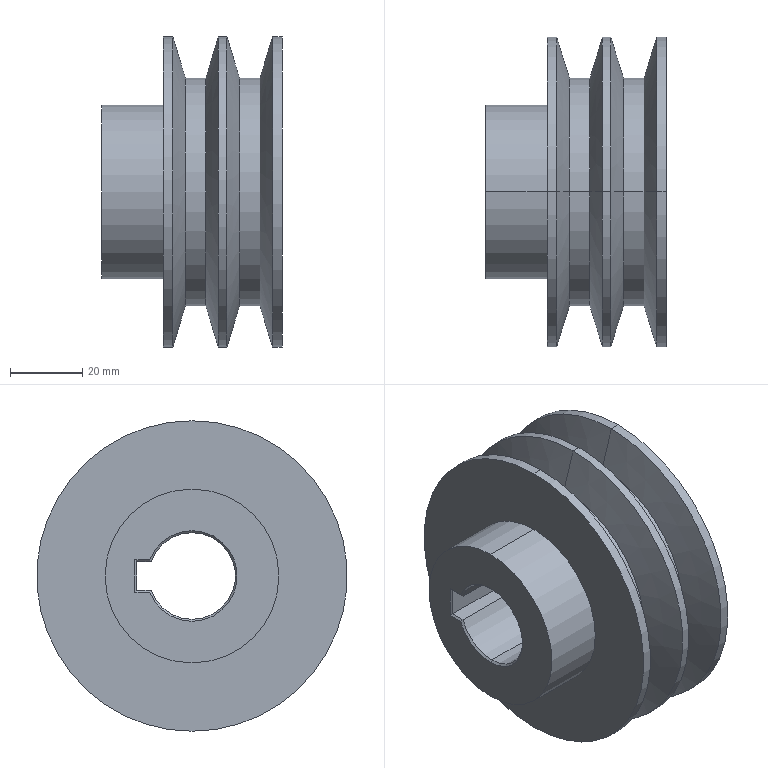Component | SolidWorks | V-beltSmallSolidWheel86x24.075x48-1 | 1 solid | 41 faces | box 50 x 86 x 86 mm | volume 148389 mm3 | cylinder 15 | cone 14 | plane 12 | commonest cylinder face diameters 86 x6 63.1 x4 24 x3 48.15 x2 | material Plain Carbon Steel
STEP:
#1=COLOUR_RGB('',0.7922,0.8196,0.9333);
#2=FILL_AREA_STYLE_COLOUR('',#1);
#3=FILL_AREA_STYLE('',(#2));
#4=SURFACE_STYLE_FILL_AREA(#3);
#5=SURFACE_SIDE_STYLE('',(#4));
#6=SURFACE_STYLE_USAGE(.BOTH.,#5);
#7=PRESENTATION_STYLE_ASSIGNMENT((#6));
#8=CARTESIAN_POINT('',(-20.311,-5.118,17.803));
#9=VERTEX_POINT('',#8);
#10=CARTESIAN_POINT('',(-20.311,-5.118,16.858));
#11=VERTEX_POINT('',#10);
#12=CARTESIAN_POINT('',(-20.311,-5.118,17.331));
#13=DIRECTION('',(1.,0.,-0.));
#14=DIRECTION('',(0.,0.,1.));
#15=AXIS2_PLACEMENT_3D('',#12,#13,#14);
#16=CIRCLE('',#15,0.4724);
#17=EDGE_CURVE('',#9,#11,#16,.T.);
#18=ORIENTED_EDGE('',*,*,#17,.F.);
#19=CARTESIAN_POINT('',(-20.29,-5.118,17.825));
#20=VERTEX_POINT('',#19);
#21=CARTESIAN_POINT('',(-20.311,-5.118,17.803));
#22=DIRECTION('',(0.7071,0.,0.7071));
#23=VECTOR('',#22,39.37);
#24=LINE('',#21,#23);
#25=EDGE_CURVE('',#9,#20,#24,.T.);
#26=ORIENTED_EDGE('',*,*,#25,.T.);
#27=CARTESIAN_POINT('',(-20.29,-5.118,16.837));
#28=VERTEX_POINT('',#27);
#29=CARTESIAN_POINT('',(-20.29,-5.118,17.331));
#30=DIRECTION('',(-1.,-0.,0.));
#31=DIRECTION('',(0.,0.,1.));
#32=AXIS2_PLACEMENT_3D('',#29,#30,#31);
#33=CIRCLE('',#32,0.4939);
#34=EDGE_CURVE('',#28,#20,#33,.T.);
#35=ORIENTED_EDGE('',*,*,#34,.F.);
#36=CARTESIAN_POINT('',(-20.311,-5.118,16.858));
#37=DIRECTION('',(0.7071,0.,-0.7071));
#38=VECTOR('',#37,39.37);
#39=LINE('',#36,#38);
#40=EDGE_CURVE('',#11,#28,#39,.T.);
#41=ORIENTED_EDGE('',*,*,#40,.F.);
#42=EDGE_LOOP('',(#18,#26,#35,#41));
#43=FACE_OUTER_BOUND('',#42,.T.);
#44=CARTESIAN_POINT('',(-20.311,-5.118,17.331));
#45=DIRECTION('',(1.,0.,-0.));
#46=DIRECTION('',(0.,0.,-1.));
#47=AXIS2_PLACEMENT_3D('',#44,#45,#46);
#48=CONICAL_SURFACE('',#47,0.4724,0.7854);
#49=ADVANCED_FACE('',(#43),#48,.F.);
#50=CARTESIAN_POINT('',(-20.311,-4.673,17.173));
#51=VERTEX_POINT('',#50);
#52=CARTESIAN_POINT('',(-20.311,-5.118,17.331));
#53=DIRECTION('',(1.,0.,-0.));
#54=DIRECTION('',(0.,0.,1.));
#55=AXIS2_PLACEMENT_3D('',#52,#53,#54);
#56=CIRCLE('',#55,0.4724);
#57=EDGE_CURVE('',#11,#51,#56,.T.);
#58=ORIENTED_EDGE('',*,*,#57,.F.);
#59=ORIENTED_EDGE('',*,*,#40,.T.);
#60=CARTESIAN_POINT('',(-20.29,-4.658,17.152));
#61=VERTEX_POINT('',#60);
#62=CARTESIAN_POINT('',(-20.29,-5.118,17.331));
#63=DIRECTION('',(-1.,-0.,0.));
#64=DIRECTION('',(0.,0.,1.));
#65=AXIS2_PLACEMENT_3D('',#62,#63,#64);
#66=CIRCLE('',#65,0.4939);
#67=EDGE_CURVE('',#61,#28,#66,.T.);
#68=ORIENTED_EDGE('',*,*,#67,.F.);
#69=CARTESIAN_POINT('',(-20.311,-4.673,17.173));
#70=CARTESIAN_POINT('',(-20.304,-4.668,17.166));
#71=CARTESIAN_POINT('',(-20.297,-4.663,17.159));
#72=CARTESIAN_POINT('',(-20.29,-4.658,17.152));
#73=B_SPLINE_CURVE_WITH_KNOTS('',3,(#69,#70,#71,#72),.UNSPECIFIED.,.F.,.F.,(4,4),(0.,0.0008589),.UNSPECIFIED.);
#74=EDGE_CURVE('',#51,#61,#73,.T.);
#75=ORIENTED_EDGE('',*,*,#74,.F.);
#76=EDGE_LOOP('',(#58,#59,#68,#75));
#77=FACE_OUTER_BOUND('',#76,.T.);
#78=CARTESIAN_POINT('',(-20.311,-5.118,17.331));
#79=DIRECTION('',(1.,0.,-0.));
#80=DIRECTION('',(0.,0.,-1.));
#81=AXIS2_PLACEMENT_3D('',#78,#79,#80);
#82=CONICAL_SURFACE('',#81,0.4724,0.7854);
#83=ADVANCED_FACE('',(#77),#82,.F.);
#84=CARTESIAN_POINT('',(-22.237,-5.118,16.858));
#85=VERTEX_POINT('',#84);
#86=CARTESIAN_POINT('',(-22.237,-5.118,17.803));
#87=VERTEX_POINT('',#86);
#88=CARTESIAN_POINT('',(-22.237,-5.118,17.331));
#89=DIRECTION('',(-1.,-0.,0.));
#90=DIRECTION('',(0.,0.,-1.));
#91=AXIS2_PLACEMENT_3D('',#88,#89,#90);
#92=CIRCLE('',#91,0.4724);
#93=EDGE_CURVE('',#85,#87,#92,.T.);
#94=ORIENTED_EDGE('',*,*,#93,.F.);
#95=CARTESIAN_POINT('',(-22.258,-5.118,16.837));
#96=VERTEX_POINT('',#95);
#97=CARTESIAN_POINT('',(-22.258,-5.118,16.837));
#98=DIRECTION('',(-0.7071,0.,-0.7071));
#99=VECTOR('',#98,39.37);
#100=LINE('',#97,#99);
#101=EDGE_CURVE('',#85,#96,#100,.T.);
#102=ORIENTED_EDGE('',*,*,#101,.T.);
#103=CARTESIAN_POINT('',(-22.258,-5.118,17.825));
#104=VERTEX_POINT('',#103);
#105=CARTESIAN_POINT('',(-22.258,-5.118,17.331));
#106=DIRECTION('',(1.,0.,-0.));
#107=DIRECTION('',(0.,0.,-1.));
#108=AXIS2_PLACEMENT_3D('',#105,#106,#107);
#109=CIRCLE('',#108,0.4939);
#110=EDGE_CURVE('',#104,#96,#109,.T.);
#111=ORIENTED_EDGE('',*,*,#110,.F.);
#112=CARTESIAN_POINT('',(-22.258,-5.118,17.825));
#113=DIRECTION('',(-0.7071,-0.,0.7071));
#114=VECTOR('',#113,39.37);
#115=LINE('',#112,#114);
#116=EDGE_CURVE('',#87,#104,#115,.T.);
#117=ORIENTED_EDGE('',*,*,#116,.F.);
#118=EDGE_LOOP('',(#94,#102,#111,#117));
#119=FACE_OUTER_BOUND('',#118,.T.);
#120=CARTESIAN_POINT('',(-22.258,-5.118,17.331));
#121=DIRECTION('',(-1.,-0.,0.));
#122=DIRECTION('',(0.,0.,1.));
#123=AXIS2_PLACEMENT_3D('',#120,#121,#122);
#124=CONICAL_SURFACE('',#123,0.4939,0.7854);
#125=ADVANCED_FACE('',(#119),#124,.F.);
#126=CARTESIAN_POINT('',(-22.237,-4.673,17.488));
#127=VERTEX_POINT('',#126);
#128=CARTESIAN_POINT('',(-22.237,-5.118,17.331));
#129=DIRECTION('',(-1.,-0.,0.));
#130=DIRECTION('',(0.,0.,-1.));
#131=AXIS2_PLACEMENT_3D('',#128,#129,#130);
#132=CIRCLE('',#131,0.4724);
#133=EDGE_CURVE('',#87,#127,#132,.T.);
#134=ORIENTED_EDGE('',*,*,#133,.F.);
#135=ORIENTED_EDGE('',*,*,#116,.T.);
#136=CARTESIAN_POINT('',(-22.258,-4.658,17.51));
#137=VERTEX_POINT('',#136);
#138=CARTESIAN_POINT('',(-22.258,-5.118,17.331));
#139=DIRECTION('',(1.,0.,-0.));
#140=DIRECTION('',(0.,0.,-1.));
#141=AXIS2_PLACEMENT_3D('',#138,#139,#140);
#142=CIRCLE('',#141,0.4939);
#143=EDGE_CURVE('',#137,#104,#142,.T.);
#144=ORIENTED_EDGE('',*,*,#143,.F.);
#145=CARTESIAN_POINT('',(-22.237,-4.673,17.488));
#146=CARTESIAN_POINT('',(-22.244,-4.668,17.496));
#147=CARTESIAN_POINT('',(-22.251,-4.663,17.503));
#148=CARTESIAN_POINT('',(-22.258,-4.658,17.51));
#149=B_SPLINE_CURVE_WITH_KNOTS('',3,(#145,#146,#147,#148),.UNSPECIFIED.,.F.,.F.,(4,4),(0.,0.0008589),.UNSPECIFIED.);
#150=EDGE_CURVE('',#127,#137,#149,.T.);
#151=ORIENTED_EDGE('',*,*,#150,.F.);
#152=EDGE_LOOP('',(#134,#135,#144,#151));
#153=FACE_OUTER_BOUND('',#152,.T.);
#154=CARTESIAN_POINT('',(-22.258,-5.118,17.331));
#155=DIRECTION('',(-1.,-0.,0.));
#156=DIRECTION('',(0.,0.,1.));
#157=AXIS2_PLACEMENT_3D('',#154,#155,#156);
#158=CONICAL_SURFACE('',#157,0.4939,0.7854);
#159=ADVANCED_FACE('',(#153),#158,.F.);
#160=CARTESIAN_POINT('',(-21.123,-5.118,16.089));
#161=VERTEX_POINT('',#160);
#162=CARTESIAN_POINT('',(-21.123,-5.118,18.573));
#163=VERTEX_POINT('',#162);
#164=CARTESIAN_POINT('',(-21.123,-5.118,17.331));
#165=DIRECTION('',(1.,0.,-0.));
#166=DIRECTION('',(0.,0.,-1.));
#167=AXIS2_PLACEMENT_3D('',#164,#165,#166);
#168=CIRCLE('',#167,1.242);
#169=EDGE_CURVE('',#161,#163,#168,.T.);
#170=ORIENTED_EDGE('',*,*,#169,.T.);
#171=CARTESIAN_POINT('',(-20.985,-5.118,19.024));
#172=VERTEX_POINT('',#171);
#173=CARTESIAN_POINT('',(-20.985,-5.118,19.024));
#174=DIRECTION('',(0.2924,0.,0.9563));
#175=VECTOR('',#174,39.37);
#176=LINE('',#173,#175);
#177=EDGE_CURVE('',#163,#172,#176,.T.);
#178=ORIENTED_EDGE('',*,*,#177,.T.);
#179=CARTESIAN_POINT('',(-20.985,-5.118,15.638));
#180=VERTEX_POINT('',#179);
#181=CARTESIAN_POINT('',(-20.985,-5.118,17.331));
#182=DIRECTION('',(1.,0.,-0.));
#183=DIRECTION('',(0.,0.,-1.));
#184=AXIS2_PLACEMENT_3D('',#181,#182,#183);
#185=CIRCLE('',#184,1.693);
#186=EDGE_CURVE('',#180,#172,#185,.T.);
#187=ORIENTED_EDGE('',*,*,#186,.F.);
#188=CARTESIAN_POINT('',(-20.985,-5.118,15.638));
#189=DIRECTION('',(0.2924,0.,-0.9563));
#190=VECTOR('',#189,39.37);
#191=LINE('',#188,#190);
#192=EDGE_CURVE('',#161,#180,#191,.T.);
#193=ORIENTED_EDGE('',*,*,#192,.F.);
#194=EDGE_LOOP('',(#170,#178,#187,#193));
#195=FACE_OUTER_BOUND('',#194,.T.);
#196=CARTESIAN_POINT('',(-20.985,-5.118,17.331));
#197=DIRECTION('',(1.,0.,-0.));
#198=DIRECTION('',(0.,0.,-1.));
#199=AXIS2_PLACEMENT_3D('',#196,#197,#198);
#200=CONICAL_SURFACE('',#199,1.693,1.274);
#201=ADVANCED_FACE('',(#195),#200,.T.);
#202=CARTESIAN_POINT('',(-21.347,-5.118,16.089));
#203=VERTEX_POINT('',#202);
#204=CARTESIAN_POINT('',(-21.347,-5.118,18.573));
#205=VERTEX_POINT('',#204);
#206=CARTESIAN_POINT('',(-21.347,-5.118,17.331));
#207=DIRECTION('',(1.,0.,-0.));
#208=DIRECTION('',(0.,0.,-1.));
#209=AXIS2_PLACEMENT_3D('',#206,#207,#208);
#210=CIRCLE('',#209,1.242);
#211=EDGE_CURVE('',#203,#205,#210,.T.);
#212=ORIENTED_EDGE('',*,*,#211,.F.);
#213=CARTESIAN_POINT('',(-21.484,-5.118,15.638));
#214=VERTEX_POINT('',#213);
#215=CARTESIAN_POINT('',(-21.347,-5.118,16.089));
#216=DIRECTION('',(-0.2924,0.,-0.9563));
#217=VECTOR('',#216,39.37);
#218=LINE('',#215,#217);
#219=EDGE_CURVE('',#203,#214,#218,.T.);
#220=ORIENTED_EDGE('',*,*,#219,.T.);
#221=CARTESIAN_POINT('',(-21.484,-5.118,19.024));
#222=VERTEX_POINT('',#221);
#223=CARTESIAN_POINT('',(-21.484,-5.118,17.331));
#224=DIRECTION('',(1.,0.,-0.));
#225=DIRECTION('',(0.,0.,-1.));
#226=AXIS2_PLACEMENT_3D('',#223,#224,#225);
#227=CIRCLE('',#226,1.693);
#228=EDGE_CURVE('',#214,#222,#227,.T.);
#229=ORIENTED_EDGE('',*,*,#228,.T.);
#230=CARTESIAN_POINT('',(-21.347,-5.118,18.573));
#231=DIRECTION('',(-0.2924,-0.,0.9563));
#232=VECTOR('',#231,39.37);
#233=LINE('',#230,#232);
#234=EDGE_CURVE('',#205,#222,#233,.T.);
#235=ORIENTED_EDGE('',*,*,#234,.F.);
#236=EDGE_LOOP('',(#212,#220,#229,#235));
#237=FACE_OUTER_BOUND('',#236,.T.);
#238=CARTESIAN_POINT('',(-21.347,-5.118,17.331));
#239=DIRECTION('',(-1.,-0.,0.));
#240=DIRECTION('',(0.,0.,1.));
#241=AXIS2_PLACEMENT_3D('',#238,#239,#240);
#242=CONICAL_SURFACE('',#241,1.242,1.274);
#243=ADVANCED_FACE('',(#237),#242,.T.);
#244=ORIENTED_EDGE('',*,*,#211,.T.);
#245=CARTESIAN_POINT('',(-21.235,-5.118,18.573));
#246=DIRECTION('',(1.,0.,-0.));
#247=VECTOR('',#246,39.37);
#248=LINE('',#245,#247);
#249=EDGE_CURVE('',#205,#163,#248,.T.);
#250=ORIENTED_EDGE('',*,*,#249,.T.);
#251=ORIENTED_EDGE('',*,*,#169,.F.);
#252=CARTESIAN_POINT('',(-21.235,-5.118,16.089));
#253=DIRECTION('',(1.,0.,-0.));
#254=VECTOR('',#253,39.37);
#255=LINE('',#252,#254);
#256=EDGE_CURVE('',#203,#161,#255,.T.);
#257=ORIENTED_EDGE('',*,*,#256,.F.);
#258=EDGE_LOOP('',(#244,#250,#251,#257));
#259=FACE_OUTER_BOUND('',#258,.T.);
#260=CARTESIAN_POINT('',(-21.235,-5.118,17.331));
#261=DIRECTION('',(1.,0.,-0.));
#262=DIRECTION('',(0.,0.,-1.));
#263=AXIS2_PLACEMENT_3D('',#260,#261,#262);
#264=CYLINDRICAL_SURFACE('',#263,1.242);
#265=ADVANCED_FACE('',(#259),#264,.T.);
#266=CARTESIAN_POINT('',(-20.532,-5.118,16.089));
#267=VERTEX_POINT('',#266);
#268=CARTESIAN_POINT('',(-20.532,-5.118,18.573));
#269=VERTEX_POINT('',#268);
#270=CARTESIAN_POINT('',(-20.532,-5.118,17.331));
#271=DIRECTION('',(1.,0.,-0.));
#272=DIRECTION('',(0.,0.,-1.));
#273=AXIS2_PLACEMENT_3D('',#270,#271,#272);
#274=CIRCLE('',#273,1.242);
#275=EDGE_CURVE('',#267,#269,#274,.T.);
#276=ORIENTED_EDGE('',*,*,#275,.T.);
#277=CARTESIAN_POINT('',(-20.395,-5.118,19.024));
#278=VERTEX_POINT('',#277);
#279=CARTESIAN_POINT('',(-20.395,-5.118,19.024));
#280=DIRECTION('',(0.2924,0.,0.9563));
#281=VECTOR('',#280,39.37);
#282=LINE('',#279,#281);
#283=EDGE_CURVE('',#269,#278,#282,.T.);
#284=ORIENTED_EDGE('',*,*,#283,.T.);
#285=CARTESIAN_POINT('',(-20.395,-5.118,15.638));
#286=VERTEX_POINT('',#285);
#287=CARTESIAN_POINT('',(-20.395,-5.118,17.331));
#288=DIRECTION('',(1.,0.,-0.));
#289=DIRECTION('',(0.,0.,-1.));
#290=AXIS2_PLACEMENT_3D('',#287,#288,#289);
#291=CIRCLE('',#290,1.693);
#292=EDGE_CURVE('',#286,#278,#291,.T.);
#293=ORIENTED_EDGE('',*,*,#292,.F.);
#294=CARTESIAN_POINT('',(-20.395,-5.118,15.638));
#295=DIRECTION('',(0.2924,0.,-0.9563));
#296=VECTOR('',#295,39.37);
#297=LINE('',#294,#296);
#298=EDGE_CURVE('',#267,#286,#297,.T.);
#299=ORIENTED_EDGE('',*,*,#298,.F.);
#300=EDGE_LOOP('',(#276,#284,#293,#299));
#301=FACE_OUTER_BOUND('',#300,.T.);
#302=CARTESIAN_POINT('',(-20.395,-5.118,17.331));
#303=DIRECTION('',(1.,0.,-0.));
#304=DIRECTION('',(0.,0.,-1.));
#305=AXIS2_PLACEMENT_3D('',#302,#303,#304);
#306=CONICAL_SURFACE('',#305,1.693,1.274);
#307=ADVANCED_FACE('',(#301),#306,.T.);
#308=CARTESIAN_POINT('',(-20.756,-5.118,16.089));
#309=VERTEX_POINT('',#308);
#310=CARTESIAN_POINT('',(-20.756,-5.118,18.573));
#311=VERTEX_POINT('',#310);
#312=CARTESIAN_POINT('',(-20.756,-5.118,17.331));
#313=DIRECTION('',(1.,0.,-0.));
#314=DIRECTION('',(0.,0.,-1.));
#315=AXIS2_PLACEMENT_3D('',#312,#313,#314);
#316=CIRCLE('',#315,1.242);
#317=EDGE_CURVE('',#309,#311,#316,.T.);
#318=ORIENTED_EDGE('',*,*,#317,.F.);
#319=CARTESIAN_POINT('',(-20.894,-5.118,15.638));
#320=VERTEX_POINT('',#319);
#321=CARTESIAN_POINT('',(-20.756,-5.118,16.089));
#322=DIRECTION('',(-0.2924,0.,-0.9563));
#323=VECTOR('',#322,39.37);
#324=LINE('',#321,#323);
#325=EDGE_CURVE('',#309,#320,#324,.T.);
#326=ORIENTED_EDGE('',*,*,#325,.T.);
#327=CARTESIAN_POINT('',(-20.894,-5.118,19.024));
#328=VERTEX_POINT('',#327);
#329=CARTESIAN_POINT('',(-20.894,-5.118,17.331));
#330=DIRECTION('',(1.,0.,-0.));
#331=DIRECTION('',(0.,0.,-1.));
#332=AXIS2_PLACEMENT_3D('',#329,#330,#331);
#333=CIRCLE('',#332,1.693);
#334=EDGE_CURVE('',#320,#328,#333,.T.);
#335=ORIENTED_EDGE('',*,*,#334,.T.);
#336=CARTESIAN_POINT('',(-20.756,-5.118,18.573));
#337=DIRECTION('',(-0.2924,-0.,0.9563));
#338=VECTOR('',#337,39.37);
#339=LINE('',#336,#338);
#340=EDGE_CURVE('',#311,#328,#339,.T.);
#341=ORIENTED_EDGE('',*,*,#340,.F.);
#342=EDGE_LOOP('',(#318,#326,#335,#341));
#343=FACE_OUTER_BOUND('',#342,.T.);
#344=CARTESIAN_POINT('',(-20.756,-5.118,17.331));
#345=DIRECTION('',(-1.,-0.,0.));
#346=DIRECTION('',(0.,0.,1.));
#347=AXIS2_PLACEMENT_3D('',#344,#345,#346);
#348=CONICAL_SURFACE('',#347,1.242,1.274);
#349=ADVANCED_FACE('',(#343),#348,.T.);
#350=ORIENTED_EDGE('',*,*,#317,.T.);
#351=CARTESIAN_POINT('',(-20.644,-5.118,18.573));
#352=DIRECTION('',(1.,0.,-0.));
#353=VECTOR('',#352,39.37);
#354=LINE('',#351,#353);
#355=EDGE_CURVE('',#311,#269,#354,.T.);
#356=ORIENTED_EDGE('',*,*,#355,.T.);
#357=ORIENTED_EDGE('',*,*,#275,.F.);
#358=CARTESIAN_POINT('',(-20.644,-5.118,16.089));
#359=DIRECTION('',(1.,0.,-0.));
#360=VECTOR('',#359,39.37);
#361=LINE('',#358,#360);
#362=EDGE_CURVE('',#309,#267,#361,.T.);
#363=ORIENTED_EDGE('',*,*,#362,.F.);
#364=EDGE_LOOP('',(#350,#356,#357,#363));
#365=FACE_OUTER_BOUND('',#364,.T.);
#366=CARTESIAN_POINT('',(-20.644,-5.118,17.331));
#367=DIRECTION('',(1.,0.,-0.));
#368=DIRECTION('',(0.,0.,-1.));
#369=AXIS2_PLACEMENT_3D('',#366,#367,#368);
#370=CYLINDRICAL_SURFACE('',#369,1.242);
#371=ADVANCED_FACE('',(#365),#370,.T.);
#372=CARTESIAN_POINT('',(-22.258,-5.118,16.383));
#373=VERTEX_POINT('',#372);
#374=CARTESIAN_POINT('',(-22.258,-5.118,18.279));
#375=VERTEX_POINT('',#374);
#376=CARTESIAN_POINT('',(-22.258,-5.118,17.331));
#377=DIRECTION('',(1.,0.,-0.));
#378=DIRECTION('',(0.,0.,-1.));
#379=AXIS2_PLACEMENT_3D('',#376,#377,#378);
#380=CIRCLE('',#379,0.9478);
#381=EDGE_CURVE('',#373,#375,#380,.T.);
#382=ORIENTED_EDGE('',*,*,#381,.T.);
#383=CARTESIAN_POINT('',(-21.589,-5.118,18.279));
#384=VERTEX_POINT('',#383);
#385=CARTESIAN_POINT('',(-20.644,-5.118,18.279));
#386=DIRECTION('',(1.,0.,-0.));
#387=VECTOR('',#386,39.37);
#388=LINE('',#385,#387);
#389=EDGE_CURVE('',#375,#384,#388,.T.);
#390=ORIENTED_EDGE('',*,*,#389,.T.);
#391=CARTESIAN_POINT('',(-21.589,-5.118,16.383));
#392=VERTEX_POINT('',#391);
#393=CARTESIAN_POINT('',(-21.589,-5.118,17.331));
#394=DIRECTION('',(1.,0.,-0.));
#395=DIRECTION('',(0.,0.,-1.));
#396=AXIS2_PLACEMENT_3D('',#393,#394,#395);
#397=CIRCLE('',#396,0.9478);
#398=EDGE_CURVE('',#392,#384,#397,.T.);
#399=ORIENTED_EDGE('',*,*,#398,.F.);
#400=CARTESIAN_POINT('',(-20.644,-5.118,16.383));
#401=DIRECTION('',(1.,0.,-0.));
#402=VECTOR('',#401,39.37);
#403=LINE('',#400,#402);
#404=EDGE_CURVE('',#373,#392,#403,.T.);
#405=ORIENTED_EDGE('',*,*,#404,.F.);
#406=EDGE_LOOP('',(#382,#390,#399,#405));
#407=FACE_OUTER_BOUND('',#406,.T.);
#408=CARTESIAN_POINT('',(-20.644,-5.118,17.331));
#409=DIRECTION('',(1.,0.,-0.));
#410=DIRECTION('',(0.,0.,-1.));
#411=AXIS2_PLACEMENT_3D('',#408,#409,#410);
#412=CYLINDRICAL_SURFACE('',#411,0.9478);
#413=ADVANCED_FACE('',(#407),#412,.T.);
#414=ORIENTED_EDGE('',*,*,#93,.T.);
#415=CARTESIAN_POINT('',(-20.644,-5.118,17.803));
#416=DIRECTION('',(1.,0.,-0.));
#417=VECTOR('',#416,39.37);
#418=LINE('',#415,#417);
#419=EDGE_CURVE('',#87,#9,#418,.T.);
#420=ORIENTED_EDGE('',*,*,#419,.T.);
#421=ORIENTED_EDGE('',*,*,#17,.T.);
#422=CARTESIAN_POINT('',(-20.644,-5.118,16.858));
#423=DIRECTION('',(1.,0.,-0.));
#424=VECTOR('',#423,39.37);
#425=LINE('',#422,#424);
#426=EDGE_CURVE('',#85,#11,#425,.T.);
#427=ORIENTED_EDGE('',*,*,#426,.F.);
#428=EDGE_LOOP('',(#414,#420,#421,#427));
#429=FACE_OUTER_BOUND('',#428,.T.);
#430=CARTESIAN_POINT('',(-20.644,-5.118,17.331));
#431=DIRECTION('',(1.,0.,-0.));
#432=DIRECTION('',(0.,0.,-1.));
#433=AXIS2_PLACEMENT_3D('',#430,#431,#432);
#434=CYLINDRICAL_SURFACE('',#433,0.4724);
#435=ADVANCED_FACE('',(#429),#434,.F.);
#436=CARTESIAN_POINT('',(-22.237,-4.673,17.173));
#437=VERTEX_POINT('',#436);
#438=CARTESIAN_POINT('',(-22.237,-5.118,17.331));
#439=DIRECTION('',(-1.,-0.,0.));
#440=DIRECTION('',(0.,0.,-1.));
#441=AXIS2_PLACEMENT_3D('',#438,#439,#440);
#442=CIRCLE('',#441,0.4724);
#443=EDGE_CURVE('',#437,#85,#442,.T.);
#444=ORIENTED_EDGE('',*,*,#443,.T.);
#445=ORIENTED_EDGE('',*,*,#426,.T.);
#446=ORIENTED_EDGE('',*,*,#57,.T.);
#447=CARTESIAN_POINT('',(-22.258,-4.673,17.173));
#448=DIRECTION('',(1.,0.,-0.));
#449=VECTOR('',#448,39.37);
#450=LINE('',#447,#449);
#451=EDGE_CURVE('',#437,#51,#450,.T.);
#452=ORIENTED_EDGE('',*,*,#451,.F.);
#453=EDGE_LOOP('',(#444,#445,#446,#452));
#454=FACE_OUTER_BOUND('',#453,.T.);
#455=CARTESIAN_POINT('',(-20.644,-5.118,17.331));
#456=DIRECTION('',(1.,0.,-0.));
#457=DIRECTION('',(0.,0.,-1.));
#458=AXIS2_PLACEMENT_3D('',#455,#456,#457);
#459=CYLINDRICAL_SURFACE('',#458,0.4724);
#460=ADVANCED_FACE('',(#454),#459,.F.);
#461=ORIENTED_EDGE('',*,*,#292,.T.);
#462=CARTESIAN_POINT('',(-20.29,-5.118,19.024));
#463=VERTEX_POINT('',#462);
#464=CARTESIAN_POINT('',(-20.644,-5.118,19.024));
#465=DIRECTION('',(1.,0.,-0.));
#466=VECTOR('',#465,39.37);
#467=LINE('',#464,#466);
#468=EDGE_CURVE('',#278,#463,#467,.T.);
#469=ORIENTED_EDGE('',*,*,#468,.T.);
#470=CARTESIAN_POINT('',(-20.29,-5.118,15.638));
#471=VERTEX_POINT('',#470);
#472=CARTESIAN_POINT('',(-20.29,-5.118,17.331));
#473=DIRECTION('',(1.,0.,-0.));
#474=DIRECTION('',(0.,0.,-1.));
#475=AXIS2_PLACEMENT_3D('',#472,#473,#474);
#476=CIRCLE('',#475,1.693);
#477=EDGE_CURVE('',#471,#463,#476,.T.);
#478=ORIENTED_EDGE('',*,*,#477,.F.);
#479=CARTESIAN_POINT('',(-20.644,-5.118,15.638));
#480=DIRECTION('',(1.,0.,-0.));
#481=VECTOR('',#480,39.37);
#482=LINE('',#479,#481);
#483=EDGE_CURVE('',#286,#471,#482,.T.);
#484=ORIENTED_EDGE('',*,*,#483,.F.);
#485=EDGE_LOOP('',(#461,#469,#478,#484));
#486=FACE_OUTER_BOUND('',#485,.T.);
#487=CARTESIAN_POINT('',(-20.644,-5.118,17.331));
#488=DIRECTION('',(1.,0.,-0.));
#489=DIRECTION('',(0.,0.,-1.));
#490=AXIS2_PLACEMENT_3D('',#487,#488,#489);
#491=CYLINDRICAL_SURFACE('',#490,1.693);
#492=ADVANCED_FACE('',(#486),#491,.T.);
#493=ORIENTED_EDGE('',*,*,#186,.T.);
#494=CARTESIAN_POINT('',(-20.644,-5.118,19.024));
#495=DIRECTION('',(1.,0.,-0.));
#496=VECTOR('',#495,39.37);
#497=LINE('',#494,#496);
#498=EDGE_CURVE('',#172,#328,#497,.T.);
#499=ORIENTED_EDGE('',*,*,#498,.T.);
#500=ORIENTED_EDGE('',*,*,#334,.F.);
#501=CARTESIAN_POINT('',(-20.644,-5.118,15.638));
#502=DIRECTION('',(1.,0.,-0.));
#503=VECTOR('',#502,39.37);
#504=LINE('',#501,#503);
#505=EDGE_CURVE('',#180,#320,#504,.T.);
#506=ORIENTED_EDGE('',*,*,#505,.F.);
#507=EDGE_LOOP('',(#493,#499,#500,#506));
#508=FACE_OUTER_BOUND('',#507,.T.);
#509=CARTESIAN_POINT('',(-20.644,-5.118,17.331));
#510=DIRECTION('',(1.,0.,-0.));
#511=DIRECTION('',(0.,0.,-1.));
#512=AXIS2_PLACEMENT_3D('',#509,#510,#511);
#513=CYLINDRICAL_SURFACE('',#512,1.693);
#514=ADVANCED_FACE('',(#508),#513,.T.);
#515=CARTESIAN_POINT('',(-21.589,-5.118,15.638));
#516=VERTEX_POINT('',#515);
#517=CARTESIAN_POINT('',(-21.589,-5.118,19.024));
#518=VERTEX_POINT('',#517);
#519=CARTESIAN_POINT('',(-21.589,-5.118,17.331));
#520=DIRECTION('',(1.,0.,-0.));
#521=DIRECTION('',(0.,0.,-1.));
#522=AXIS2_PLACEMENT_3D('',#519,#520,#521);
#523=CIRCLE('',#522,1.693);
#524=EDGE_CURVE('',#516,#518,#523,.T.);
#525=ORIENTED_EDGE('',*,*,#524,.T.);
#526=CARTESIAN_POINT('',(-20.644,-5.118,19.024));
#527=DIRECTION('',(1.,0.,-0.));
#528=VECTOR('',#527,39.37);
#529=LINE('',#526,#528);
#530=EDGE_CURVE('',#518,#222,#529,.T.);
#531=ORIENTED_EDGE('',*,*,#530,.T.);
#532=ORIENTED_EDGE('',*,*,#228,.F.);
#533=CARTESIAN_POINT('',(-20.644,-5.118,15.638));
#534=DIRECTION('',(1.,0.,-0.));
#535=VECTOR('',#534,39.37);
#536=LINE('',#533,#535);
#537=EDGE_CURVE('',#516,#214,#536,.T.);
#538=ORIENTED_EDGE('',*,*,#537,.F.);
#539=EDGE_LOOP('',(#525,#531,#532,#538));
#540=FACE_OUTER_BOUND('',#539,.T.);
#541=CARTESIAN_POINT('',(-20.644,-5.118,17.331));
#542=DIRECTION('',(1.,0.,-0.));
#543=DIRECTION('',(0.,0.,-1.));
#544=AXIS2_PLACEMENT_3D('',#541,#542,#543);
#545=CYLINDRICAL_SURFACE('',#544,1.693);
#546=ADVANCED_FACE('',(#540),#545,.T.);
#547=ORIENTED_EDGE('',*,*,#530,.F.);
#548=CARTESIAN_POINT('',(-21.589,-5.118,17.331));
#549=DIRECTION('',(1.,0.,-0.));
#550=DIRECTION('',(0.,0.,-1.));
#551=AXIS2_PLACEMENT_3D('',#548,#549,#550);
#552=CIRCLE('',#551,1.693);
#553=EDGE_CURVE('',#518,#516,#552,.T.);
#554=ORIENTED_EDGE('',*,*,#553,.T.);
#555=ORIENTED_EDGE('',*,*,#537,.T.);
#556=CARTESIAN_POINT('',(-21.484,-5.118,17.331));
#557=DIRECTION('',(1.,0.,-0.));
#558=DIRECTION('',(0.,0.,-1.));
#559=AXIS2_PLACEMENT_3D('',#556,#557,#558);
#560=CIRCLE('',#559,1.693);
#561=EDGE_CURVE('',#222,#214,#560,.T.);
#562=ORIENTED_EDGE('',*,*,#561,.F.);
#563=EDGE_LOOP('',(#547,#554,#555,#562));
#564=FACE_OUTER_BOUND('',#563,.T.);
#565=CARTESIAN_POINT('',(-20.644,-5.118,17.331));
#566=DIRECTION('',(1.,0.,-0.));
#567=DIRECTION('',(0.,0.,-1.));
#568=AXIS2_PLACEMENT_3D('',#565,#566,#567);
#569=CYLINDRICAL_SURFACE('',#568,1.693);
#570=ADVANCED_FACE('',(#564),#569,.T.);
#571=ORIENTED_EDGE('',*,*,#498,.F.);
#572=CARTESIAN_POINT('',(-20.985,-5.118,17.331));
#573=DIRECTION('',(1.,0.,-0.));
#574=DIRECTION('',(0.,0.,-1.));
#575=AXIS2_PLACEMENT_3D('',#572,#573,#574);
#576=CIRCLE('',#575,1.693);
#577=EDGE_CURVE('',#172,#180,#576,.T.);
#578=ORIENTED_EDGE('',*,*,#577,.T.);
#579=ORIENTED_EDGE('',*,*,#505,.T.);
#580=CARTESIAN_POINT('',(-20.894,-5.118,17.331));
#581=DIRECTION('',(1.,0.,-0.));
#582=DIRECTION('',(0.,0.,-1.));
#583=AXIS2_PLACEMENT_3D('',#580,#581,#582);
#584=CIRCLE('',#583,1.693);
#585=EDGE_CURVE('',#328,#320,#584,.T.);
#586=ORIENTED_EDGE('',*,*,#585,.F.);
#587=EDGE_LOOP('',(#571,#578,#579,#586));
#588=FACE_OUTER_BOUND('',#587,.T.);
#589=CARTESIAN_POINT('',(-20.644,-5.118,17.331));
#590=DIRECTION('',(1.,0.,-0.));
#591=DIRECTION('',(0.,0.,-1.));
#592=AXIS2_PLACEMENT_3D('',#589,#590,#591);
#593=CYLINDRICAL_SURFACE('',#592,1.693);
#594=ADVANCED_FACE('',(#588),#593,.T.);
#595=ORIENTED_EDGE('',*,*,#468,.F.);
#596=CARTESIAN_POINT('',(-20.395,-5.118,17.331));
#597=DIRECTION('',(1.,0.,-0.));
#598=DIRECTION('',(0.,0.,-1.));
#599=AXIS2_PLACEMENT_3D('',#596,#597,#598);
#600=CIRCLE('',#599,1.693);
#601=EDGE_CURVE('',#278,#286,#600,.T.);
#602=ORIENTED_EDGE('',*,*,#601,.T.);
#603=ORIENTED_EDGE('',*,*,#483,.T.);
#604=CARTESIAN_POINT('',(-20.29,-5.118,17.331));
#605=DIRECTION('',(1.,0.,-0.));
#606=DIRECTION('',(0.,0.,-1.));
#607=AXIS2_PLACEMENT_3D('',#604,#605,#606);
#608=CIRCLE('',#607,1.693);
#609=EDGE_CURVE('',#463,#471,#608,.T.);
#610=ORIENTED_EDGE('',*,*,#609,.F.);
#611=EDGE_LOOP('',(#595,#602,#603,#610));
#612=FACE_OUTER_BOUND('',#611,.T.);
#613=CARTESIAN_POINT('',(-20.644,-5.118,17.331));
#614=DIRECTION('',(1.,0.,-0.));
#615=DIRECTION('',(0.,0.,-1.));
#616=AXIS2_PLACEMENT_3D('',#613,#614,#615);
#617=CYLINDRICAL_SURFACE('',#616,1.693);
#618=ADVANCED_FACE('',(#612),#617,.T.);
#619=ORIENTED_EDGE('',*,*,#419,.F.);
#620=ORIENTED_EDGE('',*,*,#133,.T.);
#621=CARTESIAN_POINT('',(-20.311,-4.673,17.488));
#622=VERTEX_POINT('',#621);
#623=CARTESIAN_POINT('',(-22.258,-4.673,17.488));
#624=DIRECTION('',(1.,0.,-0.));
#625=VECTOR('',#624,39.37);
#626=LINE('',#623,#625);
#627=EDGE_CURVE('',#127,#622,#626,.T.);
#628=ORIENTED_EDGE('',*,*,#627,.T.);
#629=CARTESIAN_POINT('',(-20.311,-5.118,17.331));
#630=DIRECTION('',(1.,0.,-0.));
#631=DIRECTION('',(0.,0.,1.));
#632=AXIS2_PLACEMENT_3D('',#629,#630,#631);
#633=CIRCLE('',#632,0.4724);
#634=EDGE_CURVE('',#622,#9,#633,.T.);
#635=ORIENTED_EDGE('',*,*,#634,.T.);
#636=EDGE_LOOP('',(#619,#620,#628,#635));
#637=FACE_OUTER_BOUND('',#636,.T.);
#638=CARTESIAN_POINT('',(-20.644,-5.118,17.331));
#639=DIRECTION('',(1.,0.,-0.));
#640=DIRECTION('',(0.,0.,-1.));
#641=AXIS2_PLACEMENT_3D('',#638,#639,#640);
#642=CYLINDRICAL_SURFACE('',#641,0.4724);
#643=ADVANCED_FACE('',(#637),#642,.F.);
#644=CARTESIAN_POINT('',(-22.258,-4.494,17.152));
#645=VERTEX_POINT('',#644);
#646=CARTESIAN_POINT('',(-22.258,-4.494,17.51));
#647=VERTEX_POINT('',#646);
#648=CARTESIAN_POINT('',(-22.258,-4.494,17.331));
#649=DIRECTION('',(0.,0.,1.));
#650=VECTOR('',#649,39.37);
#651=LINE('',#648,#650);
#652=EDGE_CURVE('',#645,#647,#651,.T.);
#653=ORIENTED_EDGE('',*,*,#652,.T.);
#654=CARTESIAN_POINT('',(-22.258,-4.17,17.51));
#655=DIRECTION('',(0.,-1.,0.));
#656=VECTOR('',#655,39.37);
#657=LINE('',#654,#656);
#658=EDGE_CURVE('',#647,#137,#657,.T.);
#659=ORIENTED_EDGE('',*,*,#658,.T.);
#660=ORIENTED_EDGE('',*,*,#143,.T.);
#661=ORIENTED_EDGE('',*,*,#110,.T.);
#662=CARTESIAN_POINT('',(-22.258,-4.658,17.152));
#663=VERTEX_POINT('',#662);
#664=CARTESIAN_POINT('',(-22.258,-5.118,17.331));
#665=DIRECTION('',(1.,0.,-0.));
#666=DIRECTION('',(0.,0.,-1.));
#667=AXIS2_PLACEMENT_3D('',#664,#665,#666);
#668=CIRCLE('',#667,0.4939);
#669=EDGE_CURVE('',#96,#663,#668,.T.);
#670=ORIENTED_EDGE('',*,*,#669,.T.);
#671=CARTESIAN_POINT('',(-22.258,-4.17,17.152));
#672=DIRECTION('',(-0.,1.,0.));
#673=VECTOR('',#672,39.37);
#674=LINE('',#671,#673);
#675=EDGE_CURVE('',#663,#645,#674,.T.);
#676=ORIENTED_EDGE('',*,*,#675,.T.);
#677=EDGE_LOOP('',(#653,#659,#660,#661,#670,#676));
#678=FACE_BOUND('',#677,.T.);
#679=ORIENTED_EDGE('',*,*,#381,.F.);
#680=CARTESIAN_POINT('',(-22.258,-5.118,17.331));
#681=DIRECTION('',(1.,0.,-0.));
#682=DIRECTION('',(0.,0.,-1.));
#683=AXIS2_PLACEMENT_3D('',#680,#681,#682);
#684=CIRCLE('',#683,0.9478);
#685=EDGE_CURVE('',#375,#373,#684,.T.);
#686=ORIENTED_EDGE('',*,*,#685,.F.);
#687=EDGE_LOOP('',(#679,#686));
#688=FACE_OUTER_BOUND('',#687,.T.);
#689=CARTESIAN_POINT('',(-22.258,-4.17,17.331));
#690=DIRECTION('',(1.,0.,-0.));
#691=DIRECTION('',(-0.,0.,-1.));
#692=AXIS2_PLACEMENT_3D('',#689,#690,#691);
#693=PLANE('',#692);
#694=ADVANCED_FACE('',(#678,#688),#693,.F.);
#695=ORIENTED_EDGE('',*,*,#389,.F.);
#696=ORIENTED_EDGE('',*,*,#685,.T.);
#697=ORIENTED_EDGE('',*,*,#404,.T.);
#698=CARTESIAN_POINT('',(-21.589,-5.118,17.331));
#699=DIRECTION('',(1.,0.,-0.));
#700=DIRECTION('',(0.,0.,-1.));
#701=AXIS2_PLACEMENT_3D('',#698,#699,#700);
#702=CIRCLE('',#701,0.9478);
#703=EDGE_CURVE('',#384,#392,#702,.T.);
#704=ORIENTED_EDGE('',*,*,#703,.F.);
#705=EDGE_LOOP('',(#695,#696,#697,#704));
#706=FACE_OUTER_BOUND('',#705,.T.);
#707=CARTESIAN_POINT('',(-20.644,-5.118,17.331));
#708=DIRECTION('',(1.,0.,-0.));
#709=DIRECTION('',(0.,0.,-1.));
#710=AXIS2_PLACEMENT_3D('',#707,#708,#709);
#711=CYLINDRICAL_SURFACE('',#710,0.9478);
#712=ADVANCED_FACE('',(#706),#711,.T.);
#713=ORIENTED_EDGE('',*,*,#524,.F.);
#714=ORIENTED_EDGE('',*,*,#553,.F.);
#715=EDGE_LOOP('',(#713,#714));
#716=FACE_OUTER_BOUND('',#715,.T.);
#717=ORIENTED_EDGE('',*,*,#398,.T.);
#718=ORIENTED_EDGE('',*,*,#703,.T.);
#719=EDGE_LOOP('',(#717,#718));
#720=FACE_BOUND('',#719,.T.);
#721=CARTESIAN_POINT('',(-21.589,-3.425,17.331));
#722=DIRECTION('',(1.,0.,-0.));
#723=DIRECTION('',(-0.,0.,-1.));
#724=AXIS2_PLACEMENT_3D('',#721,#722,#723);
#725=PLANE('',#724);
#726=ADVANCED_FACE('',(#716,#720),#725,.F.);
#727=CARTESIAN_POINT('',(-20.29,-4.494,17.51));
#728=VERTEX_POINT('',#727);
#729=CARTESIAN_POINT('',(-20.29,-4.494,17.152));
#730=VERTEX_POINT('',#729);
#731=CARTESIAN_POINT('',(-20.29,-4.494,17.331));
#732=DIRECTION('',(-0.,0.,-1.));
#733=VECTOR('',#732,39.37);
#734=LINE('',#731,#733);
#735=EDGE_CURVE('',#728,#730,#734,.T.);
#736=ORIENTED_EDGE('',*,*,#735,.T.);
#737=CARTESIAN_POINT('',(-20.29,-4.646,17.152));
#738=DIRECTION('',(0.,-1.,0.));
#739=VECTOR('',#738,39.37);
#740=LINE('',#737,#739);
#741=EDGE_CURVE('',#730,#61,#740,.T.);
#742=ORIENTED_EDGE('',*,*,#741,.T.);
#743=ORIENTED_EDGE('',*,*,#67,.T.);
#744=ORIENTED_EDGE('',*,*,#34,.T.);
#745=CARTESIAN_POINT('',(-20.29,-4.658,17.51));
#746=VERTEX_POINT('',#745);
#747=CARTESIAN_POINT('',(-20.29,-5.118,17.331));
#748=DIRECTION('',(-1.,-0.,0.));
#749=DIRECTION('',(0.,0.,1.));
#750=AXIS2_PLACEMENT_3D('',#747,#748,#749);
#751=CIRCLE('',#750,0.4939);
#752=EDGE_CURVE('',#20,#746,#751,.T.);
#753=ORIENTED_EDGE('',*,*,#752,.T.);
#754=CARTESIAN_POINT('',(-20.29,-4.646,17.51));
#755=DIRECTION('',(-0.,1.,0.));
#756=VECTOR('',#755,39.37);
#757=LINE('',#754,#756);
#758=EDGE_CURVE('',#746,#728,#757,.T.);
#759=ORIENTED_EDGE('',*,*,#758,.T.);
#760=EDGE_LOOP('',(#736,#742,#743,#744,#753,#759));
#761=FACE_BOUND('',#760,.T.);
#762=ORIENTED_EDGE('',*,*,#477,.T.);
#763=ORIENTED_EDGE('',*,*,#609,.T.);
#764=EDGE_LOOP('',(#762,#763));
#765=FACE_OUTER_BOUND('',#764,.T.);
#766=CARTESIAN_POINT('',(-20.29,-4.646,17.331));
#767=DIRECTION('',(-1.,-0.,0.));
#768=DIRECTION('',(0.,0.,1.));
#769=AXIS2_PLACEMENT_3D('',#766,#767,#768);
#770=PLANE('',#769);
#771=ADVANCED_FACE('',(#761,#765),#770,.F.);
#772=ORIENTED_EDGE('',*,*,#355,.F.);
#773=CARTESIAN_POINT('',(-20.756,-5.118,17.331));
#774=DIRECTION('',(1.,0.,-0.));
#775=DIRECTION('',(0.,0.,-1.));
#776=AXIS2_PLACEMENT_3D('',#773,#774,#775);
#777=CIRCLE('',#776,1.242);
#778=EDGE_CURVE('',#311,#309,#777,.T.);
#779=ORIENTED_EDGE('',*,*,#778,.T.);
#780=ORIENTED_EDGE('',*,*,#362,.T.);
#781=CARTESIAN_POINT('',(-20.532,-5.118,17.331));
#782=DIRECTION('',(1.,0.,-0.));
#783=DIRECTION('',(0.,0.,-1.));
#784=AXIS2_PLACEMENT_3D('',#781,#782,#783);
#785=CIRCLE('',#784,1.242);
#786=EDGE_CURVE('',#269,#267,#785,.T.);
#787=ORIENTED_EDGE('',*,*,#786,.F.);
#788=EDGE_LOOP('',(#772,#779,#780,#787));
#789=FACE_OUTER_BOUND('',#788,.T.);
#790=CARTESIAN_POINT('',(-20.644,-5.118,17.331));
#791=DIRECTION('',(1.,0.,-0.));
#792=DIRECTION('',(0.,0.,-1.));
#793=AXIS2_PLACEMENT_3D('',#790,#791,#792);
#794=CYLINDRICAL_SURFACE('',#793,1.242);
#795=ADVANCED_FACE('',(#789),#794,.T.);
#796=ORIENTED_EDGE('',*,*,#325,.F.);
#797=ORIENTED_EDGE('',*,*,#778,.F.);
#798=ORIENTED_EDGE('',*,*,#340,.T.);
#799=ORIENTED_EDGE('',*,*,#585,.T.);
#800=EDGE_LOOP('',(#796,#797,#798,#799));
#801=FACE_OUTER_BOUND('',#800,.T.);
#802=CARTESIAN_POINT('',(-20.756,-5.118,17.331));
#803=DIRECTION('',(-1.,-0.,0.));
#804=DIRECTION('',(0.,0.,1.));
#805=AXIS2_PLACEMENT_3D('',#802,#803,#804);
#806=CONICAL_SURFACE('',#805,1.242,1.274);
#807=ADVANCED_FACE('',(#801),#806,.T.);
#808=ORIENTED_EDGE('',*,*,#283,.F.);
#809=ORIENTED_EDGE('',*,*,#786,.T.);
#810=ORIENTED_EDGE('',*,*,#298,.T.);
#811=ORIENTED_EDGE('',*,*,#601,.F.);
#812=EDGE_LOOP('',(#808,#809,#810,#811));
#813=FACE_OUTER_BOUND('',#812,.T.);
#814=CARTESIAN_POINT('',(-20.395,-5.118,17.331));
#815=DIRECTION('',(1.,0.,-0.));
#816=DIRECTION('',(0.,0.,-1.));
#817=AXIS2_PLACEMENT_3D('',#814,#815,#816);
#818=CONICAL_SURFACE('',#817,1.693,1.274);
#819=ADVANCED_FACE('',(#813),#818,.T.);
#820=ORIENTED_EDGE('',*,*,#249,.F.);
#821=CARTESIAN_POINT('',(-21.347,-5.118,17.331));
#822=DIRECTION('',(1.,0.,-0.));
#823=DIRECTION('',(0.,0.,-1.));
#824=AXIS2_PLACEMENT_3D('',#821,#822,#823);
#825=CIRCLE('',#824,1.242);
#826=EDGE_CURVE('',#205,#203,#825,.T.);
#827=ORIENTED_EDGE('',*,*,#826,.T.);
#828=ORIENTED_EDGE('',*,*,#256,.T.);
#829=CARTESIAN_POINT('',(-21.123,-5.118,17.331));
#830=DIRECTION('',(1.,0.,-0.));
#831=DIRECTION('',(0.,0.,-1.));
#832=AXIS2_PLACEMENT_3D('',#829,#830,#831);
#833=CIRCLE('',#832,1.242);
#834=EDGE_CURVE('',#163,#161,#833,.T.);
#835=ORIENTED_EDGE('',*,*,#834,.F.);
#836=EDGE_LOOP('',(#820,#827,#828,#835));
#837=FACE_OUTER_BOUND('',#836,.T.);
#838=CARTESIAN_POINT('',(-21.235,-5.118,17.331));
#839=DIRECTION('',(1.,0.,-0.));
#840=DIRECTION('',(0.,0.,-1.));
#841=AXIS2_PLACEMENT_3D('',#838,#839,#840);
#842=CYLINDRICAL_SURFACE('',#841,1.242);
#843=ADVANCED_FACE('',(#837),#842,.T.);
#844=ORIENTED_EDGE('',*,*,#219,.F.);
#845=ORIENTED_EDGE('',*,*,#826,.F.);
#846=ORIENTED_EDGE('',*,*,#234,.T.);
#847=ORIENTED_EDGE('',*,*,#561,.T.);
#848=EDGE_LOOP('',(#844,#845,#846,#847));
#849=FACE_OUTER_BOUND('',#848,.T.);
#850=CARTESIAN_POINT('',(-21.347,-5.118,17.331));
#851=DIRECTION('',(-1.,-0.,0.));
#852=DIRECTION('',(0.,0.,1.));
#853=AXIS2_PLACEMENT_3D('',#850,#851,#852);
#854=CONICAL_SURFACE('',#853,1.242,1.274);
#855=ADVANCED_FACE('',(#849),#854,.T.);
#856=ORIENTED_EDGE('',*,*,#177,.F.);
#857=ORIENTED_EDGE('',*,*,#834,.T.);
#858=ORIENTED_EDGE('',*,*,#192,.T.);
#859=ORIENTED_EDGE('',*,*,#577,.F.);
#860=EDGE_LOOP('',(#856,#857,#858,#859));
#861=FACE_OUTER_BOUND('',#860,.T.);
#862=CARTESIAN_POINT('',(-20.985,-5.118,17.331));
#863=DIRECTION('',(1.,0.,-0.));
#864=DIRECTION('',(0.,0.,-1.));
#865=AXIS2_PLACEMENT_3D('',#862,#863,#864);
#866=CONICAL_SURFACE('',#865,1.693,1.274);
#867=ADVANCED_FACE('',(#861),#866,.T.);
#868=ORIENTED_EDGE('',*,*,#627,.F.);
#869=CARTESIAN_POINT('',(-22.237,-4.516,17.488));
#870=VERTEX_POINT('',#869);
#871=CARTESIAN_POINT('',(-22.237,-4.673,17.488));
#872=DIRECTION('',(-0.,1.,0.));
#873=VECTOR('',#872,39.37);
#874=LINE('',#871,#873);
#875=EDGE_CURVE('',#127,#870,#874,.T.);
#876=ORIENTED_EDGE('',*,*,#875,.T.);
#877=CARTESIAN_POINT('',(-20.311,-4.516,17.488));
#878=VERTEX_POINT('',#877);
#879=CARTESIAN_POINT('',(-22.258,-4.516,17.488));
#880=DIRECTION('',(1.,0.,-0.));
#881=VECTOR('',#880,39.37);
#882=LINE('',#879,#881);
#883=EDGE_CURVE('',#870,#878,#882,.T.);
#884=ORIENTED_EDGE('',*,*,#883,.T.);
#885=CARTESIAN_POINT('',(-20.311,-4.673,17.488));
#886=DIRECTION('',(0.,-1.,0.));
#887=VECTOR('',#886,39.37);
#888=LINE('',#885,#887);
#889=EDGE_CURVE('',#878,#622,#888,.T.);
#890=ORIENTED_EDGE('',*,*,#889,.T.);
#891=EDGE_LOOP('',(#868,#876,#884,#890));
#892=FACE_OUTER_BOUND('',#891,.T.);
#893=CARTESIAN_POINT('',(-22.258,-4.673,17.488));
#894=DIRECTION('',(0.,-0.,1.));
#895=DIRECTION('',(1.,0.,-0.));
#896=AXIS2_PLACEMENT_3D('',#893,#894,#895);
#897=PLANE('',#896);
#898=ADVANCED_FACE('',(#892),#897,.F.);
#899=ORIENTED_EDGE('',*,*,#883,.F.);
#900=CARTESIAN_POINT('',(-22.237,-4.516,17.173));
#901=VERTEX_POINT('',#900);
#902=CARTESIAN_POINT('',(-22.237,-4.516,17.488));
#903=DIRECTION('',(-0.,0.,-1.));
#904=VECTOR('',#903,39.37);
#905=LINE('',#902,#904);
#906=EDGE_CURVE('',#870,#901,#905,.T.);
#907=ORIENTED_EDGE('',*,*,#906,.T.);
#908=CARTESIAN_POINT('',(-20.311,-4.516,17.173));
#909=VERTEX_POINT('',#908);
#910=CARTESIAN_POINT('',(-22.258,-4.516,17.173));
#911=DIRECTION('',(1.,0.,-0.));
#912=VECTOR('',#911,39.37);
#913=LINE('',#910,#912);
#914=EDGE_CURVE('',#901,#909,#913,.T.);
#915=ORIENTED_EDGE('',*,*,#914,.T.);
#916=CARTESIAN_POINT('',(-20.311,-4.516,17.488));
#917=DIRECTION('',(0.,0.,1.));
#918=VECTOR('',#917,39.37);
#919=LINE('',#916,#918);
#920=EDGE_CURVE('',#909,#878,#919,.T.);
#921=ORIENTED_EDGE('',*,*,#920,.T.);
#922=EDGE_LOOP('',(#899,#907,#915,#921));
#923=FACE_OUTER_BOUND('',#922,.T.);
#924=CARTESIAN_POINT('',(-22.258,-4.516,17.488));
#925=DIRECTION('',(-0.,1.,0.));
#926=DIRECTION('',(-0.,0.,-1.));
#927=AXIS2_PLACEMENT_3D('',#924,#925,#926);
#928=PLANE('',#927);
#929=ADVANCED_FACE('',(#923),#928,.F.);
#930=ORIENTED_EDGE('',*,*,#914,.F.);
#931=CARTESIAN_POINT('',(-22.237,-4.673,17.173));
#932=DIRECTION('',(0.,-1.,0.));
#933=VECTOR('',#932,39.37);
#934=LINE('',#931,#933);
#935=EDGE_CURVE('',#901,#437,#934,.T.);
#936=ORIENTED_EDGE('',*,*,#935,.T.);
#937=ORIENTED_EDGE('',*,*,#451,.T.);
#938=CARTESIAN_POINT('',(-20.311,-4.673,17.173));
#939=DIRECTION('',(-0.,1.,0.));
#940=VECTOR('',#939,39.37);
#941=LINE('',#938,#940);
#942=EDGE_CURVE('',#51,#909,#941,.T.);
#943=ORIENTED_EDGE('',*,*,#942,.T.);
#944=EDGE_LOOP('',(#930,#936,#937,#943));
#945=FACE_OUTER_BOUND('',#944,.T.);
#946=CARTESIAN_POINT('',(-22.258,-4.673,17.173));
#947=DIRECTION('',(-0.,0.,-1.));
#948=DIRECTION('',(-1.,-0.,0.));
#949=AXIS2_PLACEMENT_3D('',#946,#947,#948);
#950=PLANE('',#949);
#951=ADVANCED_FACE('',(#945),#950,.F.);
#952=CARTESIAN_POINT('',(-22.237,-4.673,17.173));
#953=CARTESIAN_POINT('',(-22.244,-4.668,17.166));
#954=CARTESIAN_POINT('',(-22.251,-4.663,17.159));
#955=CARTESIAN_POINT('',(-22.258,-4.658,17.152));
#956=B_SPLINE_CURVE_WITH_KNOTS('',3,(#952,#953,#954,#955),.UNSPECIFIED.,.F.,.F.,(4,4),(0.,0.0008589),.UNSPECIFIED.);
#957=EDGE_CURVE('',#437,#663,#956,.T.);
#958=ORIENTED_EDGE('',*,*,#957,.F.);
#959=ORIENTED_EDGE('',*,*,#935,.F.);
#960=CARTESIAN_POINT('',(-22.199,-4.554,17.212));
#961=DIRECTION('',(0.5774,-0.5774,0.5774));
#962=VECTOR('',#961,39.37);
#963=LINE('',#960,#962);
#964=EDGE_CURVE('',#645,#901,#963,.T.);
#965=ORIENTED_EDGE('',*,*,#964,.F.);
#966=ORIENTED_EDGE('',*,*,#675,.F.);
#967=EDGE_LOOP('',(#958,#959,#965,#966));
#968=FACE_OUTER_BOUND('',#967,.T.);
#969=CARTESIAN_POINT('',(-22.258,-4.17,17.152));
#970=DIRECTION('',(0.7071,0.,-0.7071));
#971=DIRECTION('',(-0.,1.,0.));
#972=AXIS2_PLACEMENT_3D('',#969,#970,#971);
#973=PLANE('',#972);
#974=ADVANCED_FACE('',(#968),#973,.F.);
#975=ORIENTED_EDGE('',*,*,#964,.T.);
#976=ORIENTED_EDGE('',*,*,#906,.F.);
#977=CARTESIAN_POINT('',(-22.366,-4.386,17.618));
#978=DIRECTION('',(0.5774,-0.5774,-0.5774));
#979=VECTOR('',#978,39.37);
#980=LINE('',#977,#979);
#981=EDGE_CURVE('',#647,#870,#980,.T.);
#982=ORIENTED_EDGE('',*,*,#981,.F.);
#983=ORIENTED_EDGE('',*,*,#652,.F.);
#984=EDGE_LOOP('',(#975,#976,#982,#983));
#985=FACE_OUTER_BOUND('',#984,.T.);
#986=CARTESIAN_POINT('',(-22.258,-4.494,17.331));
#987=DIRECTION('',(0.7071,0.7071,-0.));
#988=DIRECTION('',(0.,0.,1.));
#989=AXIS2_PLACEMENT_3D('',#986,#987,#988);
#990=PLANE('',#989);
#991=ADVANCED_FACE('',(#985),#990,.F.);
#992=ORIENTED_EDGE('',*,*,#101,.F.);
#993=ORIENTED_EDGE('',*,*,#443,.F.);
#994=ORIENTED_EDGE('',*,*,#957,.T.);
#995=ORIENTED_EDGE('',*,*,#669,.F.);
#996=EDGE_LOOP('',(#992,#993,#994,#995));
#997=FACE_OUTER_BOUND('',#996,.T.);
#998=CARTESIAN_POINT('',(-22.258,-5.118,17.331));
#999=DIRECTION('',(-1.,-0.,0.));
#1000=DIRECTION('',(0.,0.,1.));
#1001=AXIS2_PLACEMENT_3D('',#998,#999,#1000);
#1002=CONICAL_SURFACE('',#1001,0.4939,0.7854);
#1003=ADVANCED_FACE('',(#997),#1002,.F.);
#1004=ORIENTED_EDGE('',*,*,#981,.T.);
#1005=ORIENTED_EDGE('',*,*,#875,.F.);
#1006=ORIENTED_EDGE('',*,*,#150,.T.);
#1007=ORIENTED_EDGE('',*,*,#658,.F.);
#1008=EDGE_LOOP('',(#1004,#1005,#1006,#1007));
#1009=FACE_OUTER_BOUND('',#1008,.T.);
#1010=CARTESIAN_POINT('',(-22.258,-4.17,17.51));
#1011=DIRECTION('',(0.7071,0.,0.7071));
#1012=DIRECTION('',(0.,-1.,0.));
#1013=AXIS2_PLACEMENT_3D('',#1010,#1011,#1012);
#1014=PLANE('',#1013);
#1015=ADVANCED_FACE('',(#1009),#1014,.F.);
#1016=CARTESIAN_POINT('',(-20.311,-4.516,17.488));
#1017=DIRECTION('',(-0.5774,-0.5774,-0.5774));
#1018=VECTOR('',#1017,39.37);
#1019=LINE('',#1016,#1018);
#1020=EDGE_CURVE('',#728,#878,#1019,.T.);
#1021=ORIENTED_EDGE('',*,*,#1020,.F.);
#1022=ORIENTED_EDGE('',*,*,#758,.F.);
#1023=CARTESIAN_POINT('',(-20.311,-4.673,17.488));
#1024=CARTESIAN_POINT('',(-20.304,-4.668,17.496));
#1025=CARTESIAN_POINT('',(-20.297,-4.663,17.503));
#1026=CARTESIAN_POINT('',(-20.29,-4.658,17.51));
#1027=B_SPLINE_CURVE_WITH_KNOTS('',3,(#1023,#1024,#1025,#1026),.UNSPECIFIED.,.F.,.F.,(4,4),(0.,0.0008589),.UNSPECIFIED.);
#1028=EDGE_CURVE('',#622,#746,#1027,.T.);
#1029=ORIENTED_EDGE('',*,*,#1028,.F.);
#1030=ORIENTED_EDGE('',*,*,#889,.F.);
#1031=EDGE_LOOP('',(#1021,#1022,#1029,#1030));
#1032=FACE_OUTER_BOUND('',#1031,.T.);
#1033=CARTESIAN_POINT('',(-20.311,-4.673,17.488));
#1034=DIRECTION('',(-0.7071,-0.,0.7071));
#1035=DIRECTION('',(0.,-1.,0.));
#1036=AXIS2_PLACEMENT_3D('',#1033,#1034,#1035);
#1037=PLANE('',#1036);
#1038=ADVANCED_FACE('',(#1032),#1037,.F.);
#1039=ORIENTED_EDGE('',*,*,#25,.F.);
#1040=ORIENTED_EDGE('',*,*,#634,.F.);
#1041=ORIENTED_EDGE('',*,*,#1028,.T.);
#1042=ORIENTED_EDGE('',*,*,#752,.F.);
#1043=EDGE_LOOP('',(#1039,#1040,#1041,#1042));
#1044=FACE_OUTER_BOUND('',#1043,.T.);
#1045=CARTESIAN_POINT('',(-20.311,-5.118,17.331));
#1046=DIRECTION('',(1.,0.,-0.));
#1047=DIRECTION('',(0.,0.,-1.));
#1048=AXIS2_PLACEMENT_3D('',#1045,#1046,#1047);
#1049=CONICAL_SURFACE('',#1048,0.4724,0.7854);
#1050=ADVANCED_FACE('',(#1044),#1049,.F.);
#1051=ORIENTED_EDGE('',*,*,#1020,.T.);
#1052=ORIENTED_EDGE('',*,*,#920,.F.);
#1053=CARTESIAN_POINT('',(-20.364,-4.568,17.226));
#1054=DIRECTION('',(-0.5774,-0.5774,0.5774));
#1055=VECTOR('',#1054,39.37);
#1056=LINE('',#1053,#1055);
#1057=EDGE_CURVE('',#730,#909,#1056,.T.);
#1058=ORIENTED_EDGE('',*,*,#1057,.F.);
#1059=ORIENTED_EDGE('',*,*,#735,.F.);
#1060=EDGE_LOOP('',(#1051,#1052,#1058,#1059));
#1061=FACE_OUTER_BOUND('',#1060,.T.);
#1062=CARTESIAN_POINT('',(-20.311,-4.516,17.488));
#1063=DIRECTION('',(-0.7071,0.7071,0.));
#1064=DIRECTION('',(0.,0.,1.));
#1065=AXIS2_PLACEMENT_3D('',#1062,#1063,#1064);
#1066=PLANE('',#1065);
#1067=ADVANCED_FACE('',(#1061),#1066,.F.);
#1068=ORIENTED_EDGE('',*,*,#74,.T.);
#1069=ORIENTED_EDGE('',*,*,#741,.F.);
#1070=ORIENTED_EDGE('',*,*,#1057,.T.);
#1071=ORIENTED_EDGE('',*,*,#942,.F.);
#1072=EDGE_LOOP('',(#1068,#1069,#1070,#1071));
#1073=FACE_OUTER_BOUND('',#1072,.T.);
#1074=CARTESIAN_POINT('',(-20.311,-4.673,17.173));
#1075=DIRECTION('',(-0.7071,-0.,-0.7071));
#1076=DIRECTION('',(-0.,1.,0.));
#1077=AXIS2_PLACEMENT_3D('',#1074,#1075,#1076);
#1078=PLANE('',#1077);
#1079=ADVANCED_FACE('',(#1073),#1078,.F.);
#1080=CLOSED_SHELL('',(#49,#83,#125,#159,#201,#243,#265,#307,#349,#371,#413,#435,#460,#492,#514,#546,#570,#594,#618,#643,#694,#712,#726,#771,#795,#807,#819,#843,#855,#867,#898,#929,#951,#974,#991,#1003,#1015,#1038,#1050,#1067,#1079));
#1081=MANIFOLD_SOLID_BREP('',#1080);
#1082=STYLED_ITEM('',(#7),#1081);
#1083=(LENGTH_UNIT()NAMED_UNIT(*)SI_UNIT($,.METRE.));
#1084=LENGTH_MEASURE_WITH_UNIT(LENGTH_MEASURE(0.0254),#1083);
#1085=DIMENSIONAL_EXPONENTS(1.,0.,0.,0.,0.,0.,0.);
#1086=(CONVERSION_BASED_UNIT('',#1084)LENGTH_UNIT()NAMED_UNIT(#1085));
#1087=UNCERTAINTY_MEASURE_WITH_UNIT(LENGTH_MEASURE(0.00001),#1086,'','');
#1088=(NAMED_UNIT(*)PLANE_ANGLE_UNIT()SI_UNIT($,.RADIAN.));
#1089=(NAMED_UNIT(*)SI_UNIT($,.STERADIAN.)SOLID_ANGLE_UNIT());
#1090=(GEOMETRIC_REPRESENTATION_CONTEXT(3)GLOBAL_UNCERTAINTY_ASSIGNED_CONTEXT((#1087))GLOBAL_UNIT_ASSIGNED_CONTEXT((#1086,#1088,#1089))REPRESENTATION_CONTEXT('',''));
#1091=MECHANICAL_DESIGN_GEOMETRIC_PRESENTATION_REPRESENTATION('',(#1082),#1090);
#1092=PRESENTATION_LAYER_ASSIGNMENT('','',(#1082));
#1093=CARTESIAN_POINT('',(0.,0.,0.));
#1094=DIRECTION('',(0.,0.,1.));
#1095=DIRECTION('',(1.,0.,0.));
#1096=AXIS2_PLACEMENT_3D('',#1093,#1094,#1095);
#1097=(LENGTH_UNIT()NAMED_UNIT(*)SI_UNIT($,.METRE.));
#1098=LENGTH_MEASURE_WITH_UNIT(LENGTH_MEASURE(0.0254),#1097);
#1099=DIMENSIONAL_EXPONENTS(1.,0.,0.,0.,0.,0.,0.);
#1100=(CONVERSION_BASED_UNIT('',#1098)LENGTH_UNIT()NAMED_UNIT(#1099));
#1101=UNCERTAINTY_MEASURE_WITH_UNIT(LENGTH_MEASURE(0.00001),#1100,'','');
#1102=(NAMED_UNIT(*)PLANE_ANGLE_UNIT()SI_UNIT($,.RADIAN.));
#1103=(NAMED_UNIT(*)SI_UNIT($,.STERADIAN.)SOLID_ANGLE_UNIT());
#1104=(GEOMETRIC_REPRESENTATION_CONTEXT(3)GLOBAL_UNCERTAINTY_ASSIGNED_CONTEXT((#1101))GLOBAL_UNIT_ASSIGNED_CONTEXT((#1100,#1102,#1103))REPRESENTATION_CONTEXT('',''));
#1105=ADVANCED_BREP_SHAPE_REPRESENTATION('',(#1081,#1096),#1104);